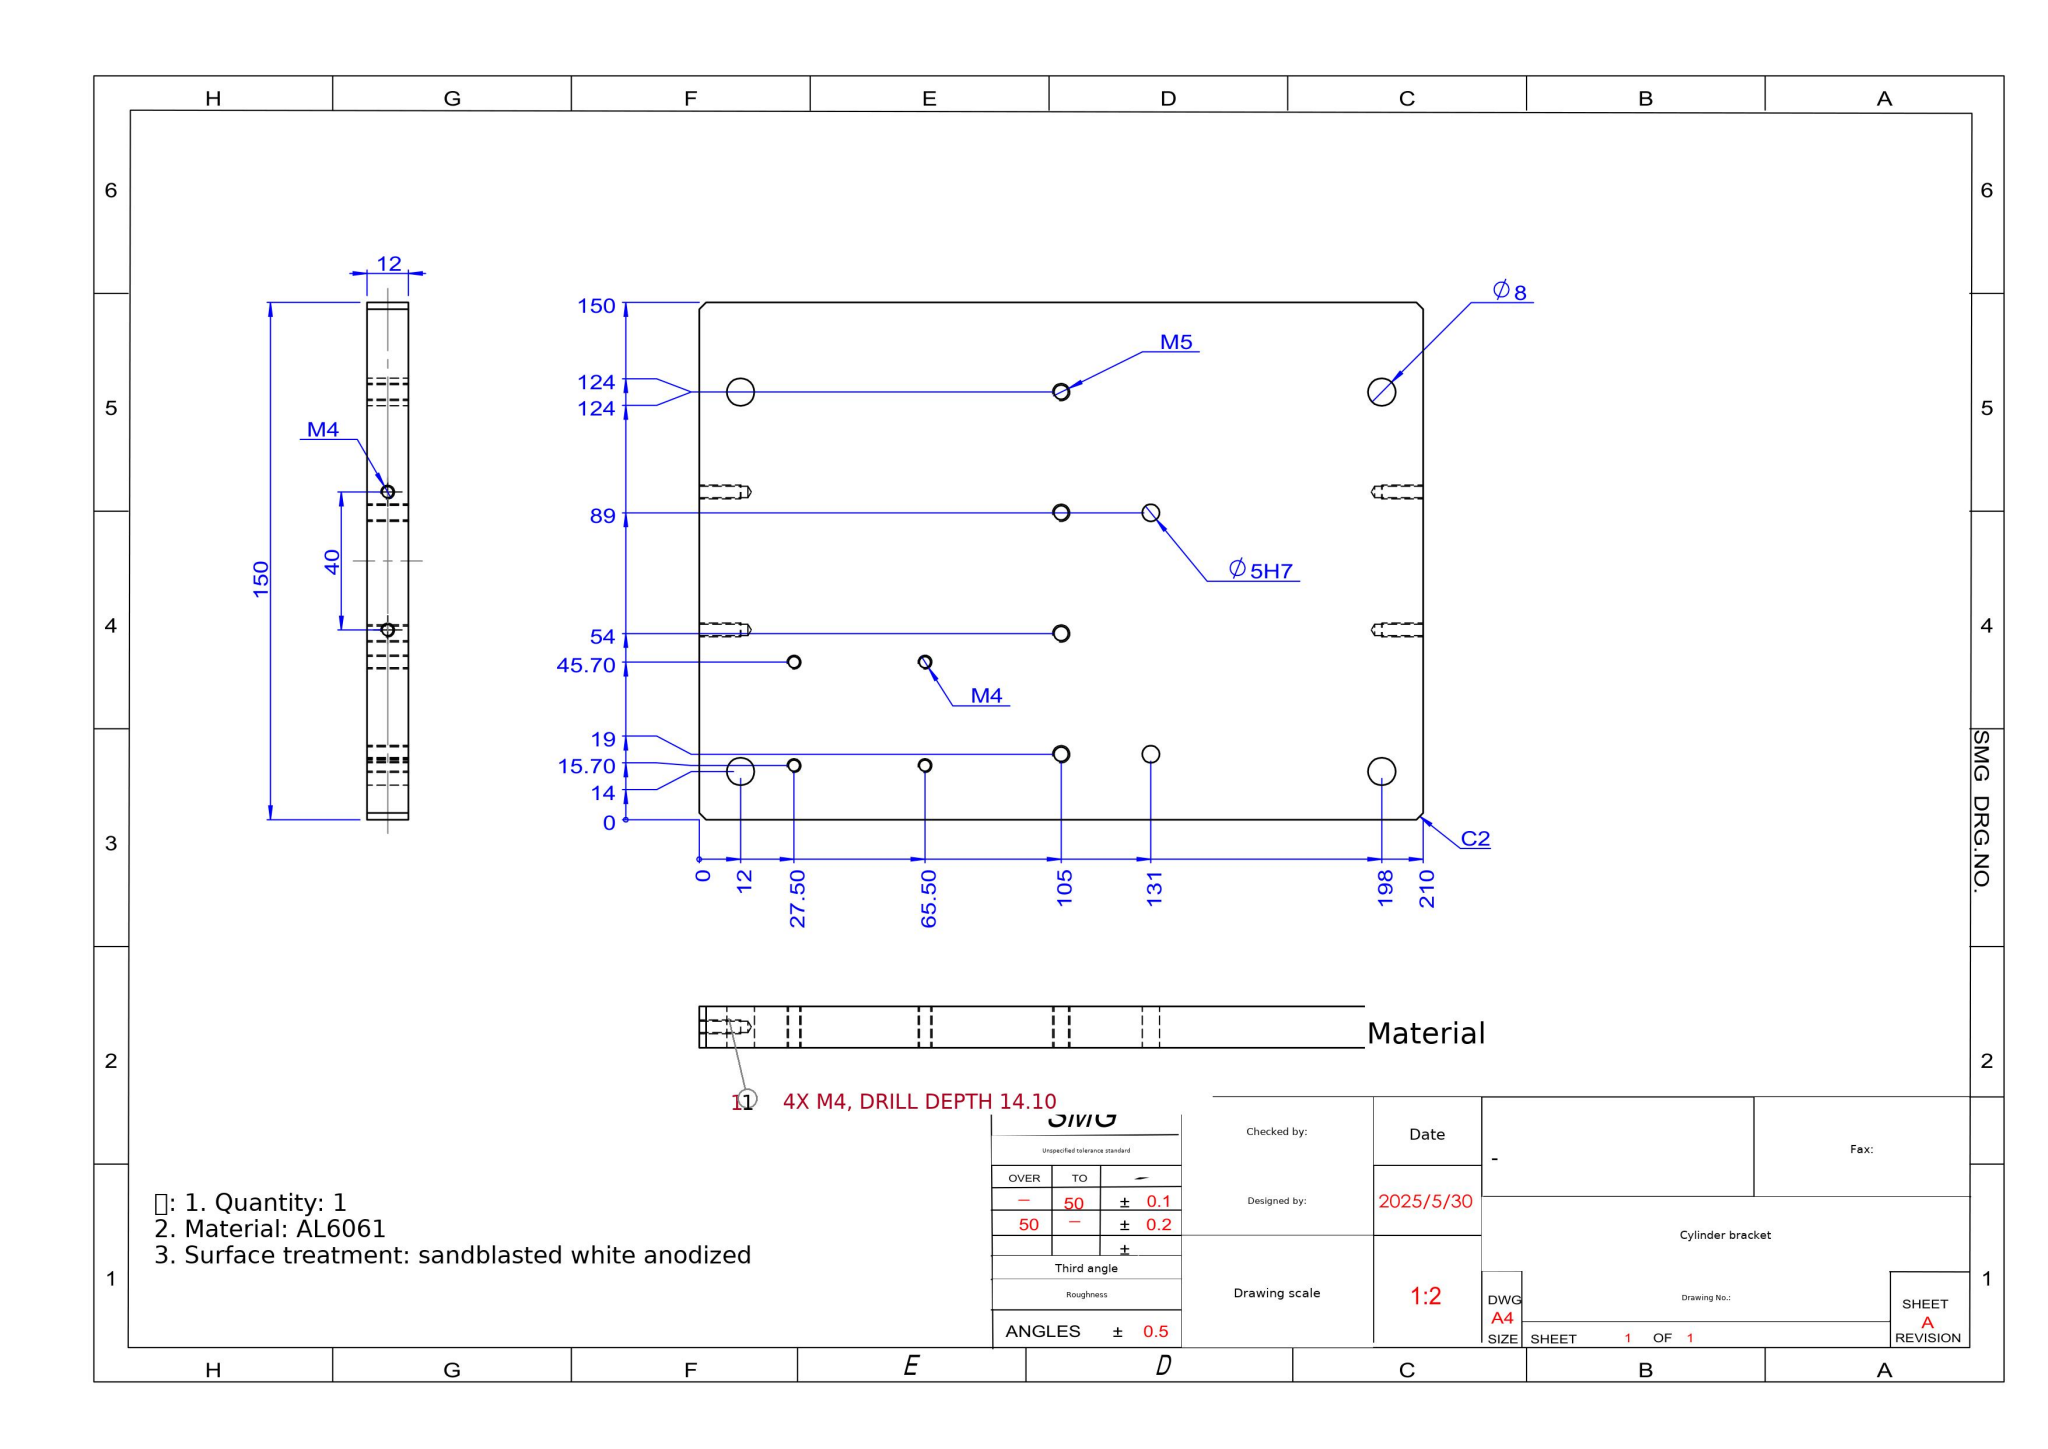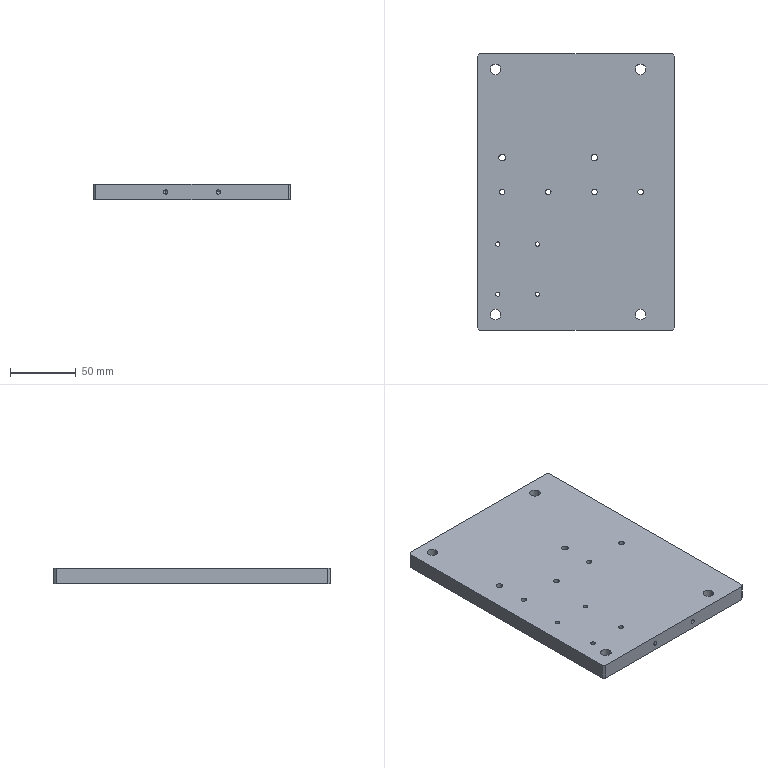Part | SolidWorks | mm | material AL6061 | 1 solid | 54 faces | box 150 x 210 x 12 mm | volume 373451 mm3 | cylinder 36 | plane 10 | cone 8 | commonest cylinder face diameters 3.3 x16 4.2 x8 8 x8 5 x4